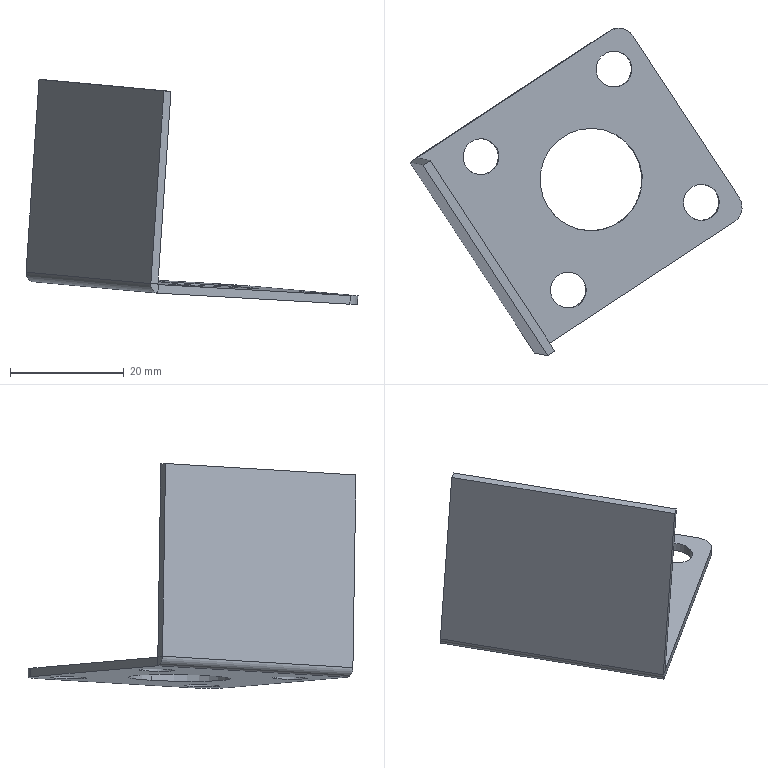Component | SolidWorks | DoorCylinderMount-1 | 1 solid | 26 faces | box 58.28 x 57.54 x 39.49 mm | volume 4144 mm3 | cylinder 14 | plane 12 | commonest cylinder face diameters 6.3 x8 18 x2 6 x2 0.2 x1 3.2 x1 | material AISI 304
STEP:
#1=CARTESIAN_POINT('',(-3.508,6.476,31.173));
#2=VERTEX_POINT('',#1);
#3=CARTESIAN_POINT('',(-3.372,6.269,31.16));
#4=VERTEX_POINT('',#3);
#5=CARTESIAN_POINT('',(-3.44,6.373,31.167));
#6=DIRECTION('',(0.0675,-0.01553,0.9976));
#7=DIRECTION('',(0.5475,-0.8353,-0.05005));
#8=AXIS2_PLACEMENT_3D('',#5,#6,#7);
#9=CIRCLE('',#8,0.124);
#10=EDGE_CURVE('',#2,#4,#9,.T.);
#11=ORIENTED_EDGE('',*,*,#10,.F.);
#12=CARTESIAN_POINT('',(-3.504,6.476,31.232));
#13=VERTEX_POINT('',#12);
#14=CARTESIAN_POINT('',(-3.504,6.476,31.232));
#15=DIRECTION('',(0.0675,-0.01553,0.9976));
#16=VECTOR('',#15,39.37);
#17=LINE('',#14,#16);
#18=EDGE_CURVE('',#2,#13,#17,.T.);
#19=ORIENTED_EDGE('',*,*,#18,.T.);
#20=CARTESIAN_POINT('',(-3.368,6.268,31.219));
#21=VERTEX_POINT('',#20);
#22=CARTESIAN_POINT('',(-3.436,6.372,31.225));
#23=DIRECTION('',(0.0675,-0.01553,0.9976));
#24=DIRECTION('',(0.5475,-0.8353,-0.05005));
#25=AXIS2_PLACEMENT_3D('',#22,#23,#24);
#26=CIRCLE('',#25,0.124);
#27=EDGE_CURVE('',#13,#21,#26,.T.);
#28=ORIENTED_EDGE('',*,*,#27,.T.);
#29=CARTESIAN_POINT('',(-3.368,6.268,31.219));
#30=DIRECTION('',(0.0675,-0.01553,0.9976));
#31=VECTOR('',#30,39.37);
#32=LINE('',#29,#31);
#33=EDGE_CURVE('',#4,#21,#32,.T.);
#34=ORIENTED_EDGE('',*,*,#33,.F.);
#35=EDGE_LOOP('',(#11,#19,#28,#34));
#36=FACE_OUTER_BOUND('',#35,.T.);
#37=CARTESIAN_POINT('',(-3.436,6.372,31.225));
#38=DIRECTION('',(0.0675,-0.01553,0.9976));
#39=DIRECTION('',(0.5475,-0.8353,-0.05005));
#40=AXIS2_PLACEMENT_3D('',#37,#38,#39);
#41=CYLINDRICAL_SURFACE('',#40,0.124);
#42=ADVANCED_FACE('',(#36),#41,.F.);
#43=CARTESIAN_POINT('',(-2.904,5.556,31.118));
#44=VERTEX_POINT('',#43);
#45=CARTESIAN_POINT('',(-2.769,5.348,31.105));
#46=VERTEX_POINT('',#45);
#47=CARTESIAN_POINT('',(-2.837,5.452,31.111));
#48=DIRECTION('',(0.0675,-0.01553,0.9976));
#49=DIRECTION('',(0.5475,-0.8353,-0.05005));
#50=AXIS2_PLACEMENT_3D('',#47,#48,#49);
#51=CIRCLE('',#50,0.124);
#52=EDGE_CURVE('',#44,#46,#51,.T.);
#53=ORIENTED_EDGE('',*,*,#52,.F.);
#54=CARTESIAN_POINT('',(-2.9,5.555,31.176));
#55=VERTEX_POINT('',#54);
#56=CARTESIAN_POINT('',(-2.9,5.555,31.176));
#57=DIRECTION('',(0.0675,-0.01553,0.9976));
#58=VECTOR('',#57,39.37);
#59=LINE('',#56,#58);
#60=EDGE_CURVE('',#44,#55,#59,.T.);
#61=ORIENTED_EDGE('',*,*,#60,.T.);
#62=CARTESIAN_POINT('',(-2.765,5.348,31.164));
#63=VERTEX_POINT('',#62);
#64=CARTESIAN_POINT('',(-2.833,5.451,31.17));
#65=DIRECTION('',(0.0675,-0.01553,0.9976));
#66=DIRECTION('',(0.5475,-0.8353,-0.05005));
#67=AXIS2_PLACEMENT_3D('',#64,#65,#66);
#68=CIRCLE('',#67,0.124);
#69=EDGE_CURVE('',#55,#63,#68,.T.);
#70=ORIENTED_EDGE('',*,*,#69,.T.);
#71=CARTESIAN_POINT('',(-2.765,5.348,31.164));
#72=DIRECTION('',(0.0675,-0.01553,0.9976));
#73=VECTOR('',#72,39.37);
#74=LINE('',#71,#73);
#75=EDGE_CURVE('',#46,#63,#74,.T.);
#76=ORIENTED_EDGE('',*,*,#75,.F.);
#77=EDGE_LOOP('',(#53,#61,#70,#76));
#78=FACE_OUTER_BOUND('',#77,.T.);
#79=CARTESIAN_POINT('',(-2.833,5.451,31.17));
#80=DIRECTION('',(0.0675,-0.01553,0.9976));
#81=DIRECTION('',(0.5475,-0.8353,-0.05005));
#82=AXIS2_PLACEMENT_3D('',#79,#80,#81);
#83=CYLINDRICAL_SURFACE('',#82,0.124);
#84=ADVANCED_FACE('',(#78),#83,.F.);
#85=CARTESIAN_POINT('',(-3.824,4.95,31.17));
#86=VERTEX_POINT('',#85);
#87=CARTESIAN_POINT('',(-3.688,4.743,31.158));
#88=VERTEX_POINT('',#87);
#89=CARTESIAN_POINT('',(-3.756,4.846,31.164));
#90=DIRECTION('',(0.0675,-0.01553,0.9976));
#91=DIRECTION('',(0.5475,-0.8353,-0.05005));
#92=AXIS2_PLACEMENT_3D('',#89,#90,#91);
#93=CIRCLE('',#92,0.124);
#94=EDGE_CURVE('',#86,#88,#93,.T.);
#95=ORIENTED_EDGE('',*,*,#94,.F.);
#96=CARTESIAN_POINT('',(-3.82,4.949,31.229));
#97=VERTEX_POINT('',#96);
#98=CARTESIAN_POINT('',(-3.82,4.949,31.229));
#99=DIRECTION('',(0.0675,-0.01553,0.9976));
#100=VECTOR('',#99,39.37);
#101=LINE('',#98,#100);
#102=EDGE_CURVE('',#86,#97,#101,.T.);
#103=ORIENTED_EDGE('',*,*,#102,.T.);
#104=CARTESIAN_POINT('',(-3.684,4.742,31.217));
#105=VERTEX_POINT('',#104);
#106=CARTESIAN_POINT('',(-3.752,4.845,31.223));
#107=DIRECTION('',(0.0675,-0.01553,0.9976));
#108=DIRECTION('',(0.5475,-0.8353,-0.05005));
#109=AXIS2_PLACEMENT_3D('',#106,#107,#108);
#110=CIRCLE('',#109,0.124);
#111=EDGE_CURVE('',#97,#105,#110,.T.);
#112=ORIENTED_EDGE('',*,*,#111,.T.);
#113=CARTESIAN_POINT('',(-3.684,4.742,31.217));
#114=DIRECTION('',(0.0675,-0.01553,0.9976));
#115=VECTOR('',#114,39.37);
#116=LINE('',#113,#115);
#117=EDGE_CURVE('',#88,#105,#116,.T.);
#118=ORIENTED_EDGE('',*,*,#117,.F.);
#119=EDGE_LOOP('',(#95,#103,#112,#118));
#120=FACE_OUTER_BOUND('',#119,.T.);
#121=CARTESIAN_POINT('',(-3.752,4.845,31.223));
#122=DIRECTION('',(0.0675,-0.01553,0.9976));
#123=DIRECTION('',(0.5475,-0.8353,-0.05005));
#124=AXIS2_PLACEMENT_3D('',#121,#122,#123);
#125=CYLINDRICAL_SURFACE('',#124,0.124);
#126=ADVANCED_FACE('',(#120),#125,.F.);
#127=CARTESIAN_POINT('',(-4.427,5.871,31.226));
#128=VERTEX_POINT('',#127);
#129=CARTESIAN_POINT('',(-4.292,5.663,31.213));
#130=VERTEX_POINT('',#129);
#131=CARTESIAN_POINT('',(-4.36,5.767,31.219));
#132=DIRECTION('',(0.0675,-0.01553,0.9976));
#133=DIRECTION('',(0.5475,-0.8353,-0.05005));
#134=AXIS2_PLACEMENT_3D('',#131,#132,#133);
#135=CIRCLE('',#134,0.124);
#136=EDGE_CURVE('',#128,#130,#135,.T.);
#137=ORIENTED_EDGE('',*,*,#136,.F.);
#138=CARTESIAN_POINT('',(-4.423,5.87,31.284));
#139=VERTEX_POINT('',#138);
#140=CARTESIAN_POINT('',(-4.423,5.87,31.284));
#141=DIRECTION('',(0.0675,-0.01553,0.9976));
#142=VECTOR('',#141,39.37);
#143=LINE('',#140,#142);
#144=EDGE_CURVE('',#128,#139,#143,.T.);
#145=ORIENTED_EDGE('',*,*,#144,.T.);
#146=CARTESIAN_POINT('',(-4.288,5.662,31.272));
#147=VERTEX_POINT('',#146);
#148=CARTESIAN_POINT('',(-4.356,5.766,31.278));
#149=DIRECTION('',(0.0675,-0.01553,0.9976));
#150=DIRECTION('',(0.5475,-0.8353,-0.05005));
#151=AXIS2_PLACEMENT_3D('',#148,#149,#150);
#152=CIRCLE('',#151,0.124);
#153=EDGE_CURVE('',#139,#147,#152,.T.);
#154=ORIENTED_EDGE('',*,*,#153,.T.);
#155=CARTESIAN_POINT('',(-4.288,5.662,31.272));
#156=DIRECTION('',(0.0675,-0.01553,0.9976));
#157=VECTOR('',#156,39.37);
#158=LINE('',#155,#157);
#159=EDGE_CURVE('',#130,#147,#158,.T.);
#160=ORIENTED_EDGE('',*,*,#159,.F.);
#161=EDGE_LOOP('',(#137,#145,#154,#160));
#162=FACE_OUTER_BOUND('',#161,.T.);
#163=CARTESIAN_POINT('',(-4.356,5.766,31.278));
#164=DIRECTION('',(0.0675,-0.01553,0.9976));
#165=DIRECTION('',(0.5475,-0.8353,-0.05005));
#166=AXIS2_PLACEMENT_3D('',#163,#164,#165);
#167=CYLINDRICAL_SURFACE('',#166,0.124);
#168=ADVANCED_FACE('',(#162),#167,.F.);
#169=CARTESIAN_POINT('',(-3.894,5.415,31.182));
#170=VERTEX_POINT('',#169);
#171=CARTESIAN_POINT('',(-3.302,5.804,31.148));
#172=VERTEX_POINT('',#171);
#173=CARTESIAN_POINT('',(-3.598,5.61,31.165));
#174=DIRECTION('',(0.0675,-0.01553,0.9976));
#175=DIRECTION('',(0.8341,0.5496,-0.04788));
#176=AXIS2_PLACEMENT_3D('',#173,#174,#175);
#177=CIRCLE('',#176,0.3543);
#178=EDGE_CURVE('',#170,#172,#177,.T.);
#179=ORIENTED_EDGE('',*,*,#178,.F.);
#180=CARTESIAN_POINT('',(-3.89,5.414,31.241));
#181=VERTEX_POINT('',#180);
#182=CARTESIAN_POINT('',(-3.89,5.414,31.241));
#183=DIRECTION('',(0.0675,-0.01553,0.9976));
#184=VECTOR('',#183,39.37);
#185=LINE('',#182,#184);
#186=EDGE_CURVE('',#170,#181,#185,.T.);
#187=ORIENTED_EDGE('',*,*,#186,.T.);
#188=CARTESIAN_POINT('',(-3.298,5.803,31.207));
#189=VERTEX_POINT('',#188);
#190=CARTESIAN_POINT('',(-3.594,5.609,31.224));
#191=DIRECTION('',(0.0675,-0.01553,0.9976));
#192=DIRECTION('',(0.8341,0.5496,-0.04788));
#193=AXIS2_PLACEMENT_3D('',#190,#191,#192);
#194=CIRCLE('',#193,0.3543);
#195=EDGE_CURVE('',#181,#189,#194,.T.);
#196=ORIENTED_EDGE('',*,*,#195,.T.);
#197=CARTESIAN_POINT('',(-3.298,5.803,31.207));
#198=DIRECTION('',(0.0675,-0.01553,0.9976));
#199=VECTOR('',#198,39.37);
#200=LINE('',#197,#199);
#201=EDGE_CURVE('',#172,#189,#200,.T.);
#202=ORIENTED_EDGE('',*,*,#201,.F.);
#203=EDGE_LOOP('',(#179,#187,#196,#202));
#204=FACE_OUTER_BOUND('',#203,.T.);
#205=CARTESIAN_POINT('',(-3.594,5.609,31.224));
#206=DIRECTION('',(0.0675,-0.01553,0.9976));
#207=DIRECTION('',(0.8341,0.5496,-0.04788));
#208=AXIS2_PLACEMENT_3D('',#205,#206,#207);
#209=CYLINDRICAL_SURFACE('',#208,0.3543);
#210=ADVANCED_FACE('',(#204),#209,.F.);
#211=CARTESIAN_POINT('',(-3.935,4.446,31.17));
#212=VERTEX_POINT('',#211);
#213=CARTESIAN_POINT('',(-2.609,5.32,31.094));
#214=VERTEX_POINT('',#213);
#215=CARTESIAN_POINT('',(-2.51,5.385,31.088));
#216=DIRECTION('',(0.8341,0.5496,-0.04788));
#217=VECTOR('',#216,39.37);
#218=LINE('',#215,#217);
#219=EDGE_CURVE('',#212,#214,#218,.T.);
#220=ORIENTED_EDGE('',*,*,#219,.T.);
#221=CARTESIAN_POINT('',(-2.605,5.319,31.153));
#222=VERTEX_POINT('',#221);
#223=CARTESIAN_POINT('',(-2.605,5.319,31.153));
#224=DIRECTION('',(0.0675,-0.01553,0.9976));
#225=VECTOR('',#224,39.37);
#226=LINE('',#223,#225);
#227=EDGE_CURVE('',#214,#222,#226,.T.);
#228=ORIENTED_EDGE('',*,*,#227,.T.);
#229=CARTESIAN_POINT('',(-3.931,4.445,31.229));
#230=VERTEX_POINT('',#229);
#231=CARTESIAN_POINT('',(-2.506,5.384,31.147));
#232=DIRECTION('',(0.8341,0.5496,-0.04788));
#233=VECTOR('',#232,39.37);
#234=LINE('',#231,#233);
#235=EDGE_CURVE('',#230,#222,#234,.T.);
#236=ORIENTED_EDGE('',*,*,#235,.F.);
#237=CARTESIAN_POINT('',(-3.931,4.445,31.229));
#238=DIRECTION('',(0.0675,-0.01553,0.9976));
#239=VECTOR('',#238,39.37);
#240=LINE('',#237,#239);
#241=EDGE_CURVE('',#212,#230,#240,.T.);
#242=ORIENTED_EDGE('',*,*,#241,.F.);
#243=EDGE_LOOP('',(#220,#228,#236,#242));
#244=FACE_OUTER_BOUND('',#243,.T.);
#245=CARTESIAN_POINT('',(-2.506,5.384,31.147));
#246=DIRECTION('',(-0.5475,0.8353,0.05005));
#247=DIRECTION('',(0.8341,0.5496,-0.04788));
#248=AXIS2_PLACEMENT_3D('',#245,#246,#247);
#249=PLANE('',#248);
#250=ADVANCED_FACE('',(#244),#249,.F.);
#251=CARTESIAN_POINT('',(-3.308,6.601,31.161));
#252=VERTEX_POINT('',#251);
#253=CARTESIAN_POINT('',(-2.575,5.483,31.094));
#254=VERTEX_POINT('',#253);
#255=CARTESIAN_POINT('',(-3.372,6.7,31.167));
#256=DIRECTION('',(0.5475,-0.8353,-0.05005));
#257=VECTOR('',#256,39.37);
#258=LINE('',#255,#257);
#259=EDGE_CURVE('',#252,#254,#258,.T.);
#260=ORIENTED_EDGE('',*,*,#259,.F.);
#261=CARTESIAN_POINT('',(-3.304,6.6,31.22));
#262=VERTEX_POINT('',#261);
#263=CARTESIAN_POINT('',(-3.304,6.6,31.22));
#264=DIRECTION('',(0.0675,-0.01553,0.9976));
#265=VECTOR('',#264,39.37);
#266=LINE('',#263,#265);
#267=EDGE_CURVE('',#252,#262,#266,.T.);
#268=ORIENTED_EDGE('',*,*,#267,.T.);
#269=CARTESIAN_POINT('',(-2.571,5.482,31.153));
#270=VERTEX_POINT('',#269);
#271=CARTESIAN_POINT('',(-3.368,6.699,31.226));
#272=DIRECTION('',(0.5475,-0.8353,-0.05005));
#273=VECTOR('',#272,39.37);
#274=LINE('',#271,#273);
#275=EDGE_CURVE('',#262,#270,#274,.T.);
#276=ORIENTED_EDGE('',*,*,#275,.T.);
#277=CARTESIAN_POINT('',(-2.571,5.482,31.153));
#278=DIRECTION('',(-0.0675,0.01553,-0.9976));
#279=VECTOR('',#278,39.37);
#280=LINE('',#277,#279);
#281=EDGE_CURVE('',#270,#254,#280,.T.);
#282=ORIENTED_EDGE('',*,*,#281,.T.);
#283=EDGE_LOOP('',(#260,#268,#276,#282));
#284=FACE_OUTER_BOUND('',#283,.T.);
#285=CARTESIAN_POINT('',(-3.368,6.699,31.226));
#286=DIRECTION('',(0.8341,0.5496,-0.04788));
#287=DIRECTION('',(0.5475,-0.8353,-0.05005));
#288=AXIS2_PLACEMENT_3D('',#285,#286,#287);
#289=PLANE('',#288);
#290=ADVANCED_FACE('',(#284),#289,.T.);
#291=CARTESIAN_POINT('',(-4.794,5.76,31.308));
#292=VERTEX_POINT('',#291);
#293=CARTESIAN_POINT('',(-3.467,6.634,31.232));
#294=VERTEX_POINT('',#293);
#295=CARTESIAN_POINT('',(-3.368,6.699,31.226));
#296=DIRECTION('',(0.8341,0.5496,-0.04788));
#297=VECTOR('',#296,39.37);
#298=LINE('',#295,#297);
#299=EDGE_CURVE('',#292,#294,#298,.T.);
#300=ORIENTED_EDGE('',*,*,#299,.T.);
#301=CARTESIAN_POINT('',(-3.471,6.635,31.173));
#302=VERTEX_POINT('',#301);
#303=CARTESIAN_POINT('',(-3.467,6.634,31.232));
#304=DIRECTION('',(-0.0675,0.01553,-0.9976));
#305=VECTOR('',#304,39.37);
#306=LINE('',#303,#305);
#307=EDGE_CURVE('',#294,#302,#306,.T.);
#308=ORIENTED_EDGE('',*,*,#307,.T.);
#309=CARTESIAN_POINT('',(-4.798,5.761,31.249));
#310=VERTEX_POINT('',#309);
#311=CARTESIAN_POINT('',(-3.372,6.7,31.167));
#312=DIRECTION('',(0.8341,0.5496,-0.04788));
#313=VECTOR('',#312,39.37);
#314=LINE('',#311,#313);
#315=EDGE_CURVE('',#310,#302,#314,.T.);
#316=ORIENTED_EDGE('',*,*,#315,.F.);
#317=CARTESIAN_POINT('',(-4.794,5.76,31.308));
#318=DIRECTION('',(0.0675,-0.01553,0.9976));
#319=VECTOR('',#318,39.37);
#320=LINE('',#317,#319);
#321=EDGE_CURVE('',#310,#292,#320,.T.);
#322=ORIENTED_EDGE('',*,*,#321,.T.);
#323=EDGE_LOOP('',(#300,#308,#316,#322));
#324=FACE_OUTER_BOUND('',#323,.T.);
#325=CARTESIAN_POINT('',(-3.368,6.699,31.226));
#326=DIRECTION('',(-0.5475,0.8353,0.05005));
#327=DIRECTION('',(0.8341,0.5496,-0.04788));
#328=AXIS2_PLACEMENT_3D('',#325,#326,#327);
#329=PLANE('',#328);
#330=ADVANCED_FACE('',(#324),#329,.T.);
#331=ORIENTED_EDGE('',*,*,#321,.F.);
#332=CARTESIAN_POINT('',(-4.846,5.725,31.315));
#333=VERTEX_POINT('',#332);
#334=CARTESIAN_POINT('',(-4.793,5.76,31.312));
#335=DIRECTION('',(-0.5475,0.8353,0.05005));
#336=DIRECTION('',(0.0675,-0.01553,0.9976));
#337=AXIS2_PLACEMENT_3D('',#334,#335,#336);
#338=CIRCLE('',#337,0.06299);
#339=EDGE_CURVE('',#310,#333,#338,.T.);
#340=ORIENTED_EDGE('',*,*,#339,.T.);
#341=CARTESIAN_POINT('',(-4.797,5.758,31.312));
#342=VERTEX_POINT('',#341);
#343=CARTESIAN_POINT('',(-4.797,5.758,31.312));
#344=DIRECTION('',(0.8341,0.5496,-0.04788));
#345=VECTOR('',#344,39.37);
#346=LINE('',#343,#345);
#347=EDGE_CURVE('',#333,#342,#346,.T.);
#348=ORIENTED_EDGE('',*,*,#347,.T.);
#349=CARTESIAN_POINT('',(-4.793,5.76,31.312));
#350=DIRECTION('',(-0.5475,0.8353,0.05005));
#351=DIRECTION('',(-0.0675,0.01553,-0.9976));
#352=AXIS2_PLACEMENT_3D('',#349,#350,#351);
#353=CIRCLE('',#352,0.003937);
#354=EDGE_CURVE('',#292,#342,#353,.T.);
#355=ORIENTED_EDGE('',*,*,#354,.F.);
#356=EDGE_LOOP('',(#331,#340,#348,#355));
#357=FACE_OUTER_BOUND('',#356,.T.);
#358=CARTESIAN_POINT('',(-4.793,5.76,31.312));
#359=DIRECTION('',(-0.5475,0.8353,0.05005));
#360=DIRECTION('',(0.0675,-0.01553,0.9976));
#361=AXIS2_PLACEMENT_3D('',#358,#359,#360);
#362=PLANE('',#361);
#363=ADVANCED_FACE('',(#357),#362,.T.);
#364=ORIENTED_EDGE('',*,*,#347,.F.);
#365=CARTESIAN_POINT('',(-4.756,5.705,32.646));
#366=VERTEX_POINT('',#365);
#367=CARTESIAN_POINT('',(-4.846,5.725,31.311));
#368=DIRECTION('',(-0.0675,0.01553,-0.9976));
#369=VECTOR('',#368,39.37);
#370=LINE('',#367,#369);
#371=EDGE_CURVE('',#366,#333,#370,.T.);
#372=ORIENTED_EDGE('',*,*,#371,.F.);
#373=CARTESIAN_POINT('',(-4.706,5.737,32.643));
#374=VERTEX_POINT('',#373);
#375=CARTESIAN_POINT('',(-4.706,5.737,32.643));
#376=DIRECTION('',(0.8341,0.5496,-0.04788));
#377=VECTOR('',#376,39.37);
#378=LINE('',#375,#377);
#379=EDGE_CURVE('',#366,#374,#378,.T.);
#380=ORIENTED_EDGE('',*,*,#379,.T.);
#381=CARTESIAN_POINT('',(-4.797,5.758,31.308));
#382=DIRECTION('',(-0.0675,0.01553,-0.9976));
#383=VECTOR('',#382,39.37);
#384=LINE('',#381,#383);
#385=EDGE_CURVE('',#374,#342,#384,.T.);
#386=ORIENTED_EDGE('',*,*,#385,.T.);
#387=EDGE_LOOP('',(#364,#372,#380,#386));
#388=FACE_OUTER_BOUND('',#387,.T.);
#389=CARTESIAN_POINT('',(-4.797,5.758,31.308));
#390=DIRECTION('',(-0.5475,0.8353,0.05005));
#391=DIRECTION('',(-0.0675,0.01553,-0.9976));
#392=AXIS2_PLACEMENT_3D('',#389,#390,#391);
#393=PLANE('',#392);
#394=ADVANCED_FACE('',(#388),#393,.T.);
#395=ORIENTED_EDGE('',*,*,#379,.F.);
#396=CARTESIAN_POINT('',(-3.893,4.389,32.567));
#397=VERTEX_POINT('',#396);
#398=CARTESIAN_POINT('',(-4.756,5.705,32.646));
#399=DIRECTION('',(0.5475,-0.8353,-0.05005));
#400=VECTOR('',#399,39.37);
#401=LINE('',#398,#400);
#402=EDGE_CURVE('',#366,#397,#401,.T.);
#403=ORIENTED_EDGE('',*,*,#402,.T.);
#404=CARTESIAN_POINT('',(-3.844,4.422,32.565));
#405=VERTEX_POINT('',#404);
#406=CARTESIAN_POINT('',(-3.844,4.422,32.565));
#407=DIRECTION('',(0.8341,0.5496,-0.04788));
#408=VECTOR('',#407,39.37);
#409=LINE('',#406,#408);
#410=EDGE_CURVE('',#397,#405,#409,.T.);
#411=ORIENTED_EDGE('',*,*,#410,.T.);
#412=CARTESIAN_POINT('',(-4.706,5.737,32.643));
#413=DIRECTION('',(0.5475,-0.8353,-0.05005));
#414=VECTOR('',#413,39.37);
#415=LINE('',#412,#414);
#416=EDGE_CURVE('',#374,#405,#415,.T.);
#417=ORIENTED_EDGE('',*,*,#416,.F.);
#418=EDGE_LOOP('',(#395,#403,#411,#417));
#419=FACE_OUTER_BOUND('',#418,.T.);
#420=CARTESIAN_POINT('',(-4.706,5.737,32.643));
#421=DIRECTION('',(-0.0675,0.01553,-0.9976));
#422=DIRECTION('',(0.5475,-0.8353,-0.05005));
#423=AXIS2_PLACEMENT_3D('',#420,#421,#422);
#424=PLANE('',#423);
#425=ADVANCED_FACE('',(#419),#424,.F.);
#426=ORIENTED_EDGE('',*,*,#410,.F.);
#427=CARTESIAN_POINT('',(-3.984,4.41,31.236));
#428=VERTEX_POINT('',#427);
#429=CARTESIAN_POINT('',(-3.984,4.41,31.232));
#430=DIRECTION('',(-0.0675,0.01553,-0.9976));
#431=VECTOR('',#430,39.37);
#432=LINE('',#429,#431);
#433=EDGE_CURVE('',#397,#428,#432,.T.);
#434=ORIENTED_EDGE('',*,*,#433,.T.);
#435=CARTESIAN_POINT('',(-3.934,4.442,31.233));
#436=VERTEX_POINT('',#435);
#437=CARTESIAN_POINT('',(-3.934,4.442,31.233));
#438=DIRECTION('',(0.8341,0.5496,-0.04788));
#439=VECTOR('',#438,39.37);
#440=LINE('',#437,#439);
#441=EDGE_CURVE('',#428,#436,#440,.T.);
#442=ORIENTED_EDGE('',*,*,#441,.T.);
#443=CARTESIAN_POINT('',(-3.935,4.442,31.229));
#444=DIRECTION('',(-0.0675,0.01553,-0.9976));
#445=VECTOR('',#444,39.37);
#446=LINE('',#443,#445);
#447=EDGE_CURVE('',#405,#436,#446,.T.);
#448=ORIENTED_EDGE('',*,*,#447,.F.);
#449=EDGE_LOOP('',(#426,#434,#442,#448));
#450=FACE_OUTER_BOUND('',#449,.T.);
#451=CARTESIAN_POINT('',(-3.935,4.442,31.229));
#452=DIRECTION('',(-0.5475,0.8353,0.05005));
#453=DIRECTION('',(-0.0675,0.01553,-0.9976));
#454=AXIS2_PLACEMENT_3D('',#451,#452,#453);
#455=PLANE('',#454);
#456=ADVANCED_FACE('',(#450),#455,.F.);
#457=ORIENTED_EDGE('',*,*,#186,.F.);
#458=CARTESIAN_POINT('',(-3.598,5.61,31.165));
#459=DIRECTION('',(0.0675,-0.01553,0.9976));
#460=DIRECTION('',(0.8341,0.5496,-0.04788));
#461=AXIS2_PLACEMENT_3D('',#458,#459,#460);
#462=CIRCLE('',#461,0.3543);
#463=EDGE_CURVE('',#172,#170,#462,.T.);
#464=ORIENTED_EDGE('',*,*,#463,.F.);
#465=ORIENTED_EDGE('',*,*,#201,.T.);
#466=CARTESIAN_POINT('',(-3.594,5.609,31.224));
#467=DIRECTION('',(0.0675,-0.01553,0.9976));
#468=DIRECTION('',(0.8341,0.5496,-0.04788));
#469=AXIS2_PLACEMENT_3D('',#466,#467,#468);
#470=CIRCLE('',#469,0.3543);
#471=EDGE_CURVE('',#189,#181,#470,.T.);
#472=ORIENTED_EDGE('',*,*,#471,.T.);
#473=EDGE_LOOP('',(#457,#464,#465,#472));
#474=FACE_OUTER_BOUND('',#473,.T.);
#475=CARTESIAN_POINT('',(-3.594,5.609,31.224));
#476=DIRECTION('',(0.0675,-0.01553,0.9976));
#477=DIRECTION('',(0.8341,0.5496,-0.04788));
#478=AXIS2_PLACEMENT_3D('',#475,#476,#477);
#479=CYLINDRICAL_SURFACE('',#478,0.3543);
#480=ADVANCED_FACE('',(#474),#479,.F.);
#481=ORIENTED_EDGE('',*,*,#144,.F.);
#482=CARTESIAN_POINT('',(-4.36,5.767,31.219));
#483=DIRECTION('',(0.0675,-0.01553,0.9976));
#484=DIRECTION('',(0.5475,-0.8353,-0.05005));
#485=AXIS2_PLACEMENT_3D('',#482,#483,#484);
#486=CIRCLE('',#485,0.124);
#487=EDGE_CURVE('',#130,#128,#486,.T.);
#488=ORIENTED_EDGE('',*,*,#487,.F.);
#489=ORIENTED_EDGE('',*,*,#159,.T.);
#490=CARTESIAN_POINT('',(-4.356,5.766,31.278));
#491=DIRECTION('',(0.0675,-0.01553,0.9976));
#492=DIRECTION('',(0.5475,-0.8353,-0.05005));
#493=AXIS2_PLACEMENT_3D('',#490,#491,#492);
#494=CIRCLE('',#493,0.124);
#495=EDGE_CURVE('',#147,#139,#494,.T.);
#496=ORIENTED_EDGE('',*,*,#495,.T.);
#497=EDGE_LOOP('',(#481,#488,#489,#496));
#498=FACE_OUTER_BOUND('',#497,.T.);
#499=CARTESIAN_POINT('',(-4.356,5.766,31.278));
#500=DIRECTION('',(0.0675,-0.01553,0.9976));
#501=DIRECTION('',(0.5475,-0.8353,-0.05005));
#502=AXIS2_PLACEMENT_3D('',#499,#500,#501);
#503=CYLINDRICAL_SURFACE('',#502,0.124);
#504=ADVANCED_FACE('',(#498),#503,.F.);
#505=ORIENTED_EDGE('',*,*,#102,.F.);
#506=CARTESIAN_POINT('',(-3.756,4.846,31.164));
#507=DIRECTION('',(0.0675,-0.01553,0.9976));
#508=DIRECTION('',(0.5475,-0.8353,-0.05005));
#509=AXIS2_PLACEMENT_3D('',#506,#507,#508);
#510=CIRCLE('',#509,0.124);
#511=EDGE_CURVE('',#88,#86,#510,.T.);
#512=ORIENTED_EDGE('',*,*,#511,.F.);
#513=ORIENTED_EDGE('',*,*,#117,.T.);
#514=CARTESIAN_POINT('',(-3.752,4.845,31.223));
#515=DIRECTION('',(0.0675,-0.01553,0.9976));
#516=DIRECTION('',(0.5475,-0.8353,-0.05005));
#517=AXIS2_PLACEMENT_3D('',#514,#515,#516);
#518=CIRCLE('',#517,0.124);
#519=EDGE_CURVE('',#105,#97,#518,.T.);
#520=ORIENTED_EDGE('',*,*,#519,.T.);
#521=EDGE_LOOP('',(#505,#512,#513,#520));
#522=FACE_OUTER_BOUND('',#521,.T.);
#523=CARTESIAN_POINT('',(-3.752,4.845,31.223));
#524=DIRECTION('',(0.0675,-0.01553,0.9976));
#525=DIRECTION('',(0.5475,-0.8353,-0.05005));
#526=AXIS2_PLACEMENT_3D('',#523,#524,#525);
#527=CYLINDRICAL_SURFACE('',#526,0.124);
#528=ADVANCED_FACE('',(#522),#527,.F.);
#529=ORIENTED_EDGE('',*,*,#60,.F.);
#530=CARTESIAN_POINT('',(-2.837,5.452,31.111));
#531=DIRECTION('',(0.0675,-0.01553,0.9976));
#532=DIRECTION('',(0.5475,-0.8353,-0.05005));
#533=AXIS2_PLACEMENT_3D('',#530,#531,#532);
#534=CIRCLE('',#533,0.124);
#535=EDGE_CURVE('',#46,#44,#534,.T.);
#536=ORIENTED_EDGE('',*,*,#535,.F.);
#537=ORIENTED_EDGE('',*,*,#75,.T.);
#538=CARTESIAN_POINT('',(-2.833,5.451,31.17));
#539=DIRECTION('',(0.0675,-0.01553,0.9976));
#540=DIRECTION('',(0.5475,-0.8353,-0.05005));
#541=AXIS2_PLACEMENT_3D('',#538,#539,#540);
#542=CIRCLE('',#541,0.124);
#543=EDGE_CURVE('',#63,#55,#542,.T.);
#544=ORIENTED_EDGE('',*,*,#543,.T.);
#545=EDGE_LOOP('',(#529,#536,#537,#544));
#546=FACE_OUTER_BOUND('',#545,.T.);
#547=CARTESIAN_POINT('',(-2.833,5.451,31.17));
#548=DIRECTION('',(0.0675,-0.01553,0.9976));
#549=DIRECTION('',(0.5475,-0.8353,-0.05005));
#550=AXIS2_PLACEMENT_3D('',#547,#548,#549);
#551=CYLINDRICAL_SURFACE('',#550,0.124);
#552=ADVANCED_FACE('',(#546),#551,.F.);
#553=ORIENTED_EDGE('',*,*,#18,.F.);
#554=CARTESIAN_POINT('',(-3.44,6.373,31.167));
#555=DIRECTION('',(0.0675,-0.01553,0.9976));
#556=DIRECTION('',(0.5475,-0.8353,-0.05005));
#557=AXIS2_PLACEMENT_3D('',#554,#555,#556);
#558=CIRCLE('',#557,0.124);
#559=EDGE_CURVE('',#4,#2,#558,.T.);
#560=ORIENTED_EDGE('',*,*,#559,.F.);
#561=ORIENTED_EDGE('',*,*,#33,.T.);
#562=CARTESIAN_POINT('',(-3.436,6.372,31.225));
#563=DIRECTION('',(0.0675,-0.01553,0.9976));
#564=DIRECTION('',(0.5475,-0.8353,-0.05005));
#565=AXIS2_PLACEMENT_3D('',#562,#563,#564);
#566=CIRCLE('',#565,0.124);
#567=EDGE_CURVE('',#21,#13,#566,.T.);
#568=ORIENTED_EDGE('',*,*,#567,.T.);
#569=EDGE_LOOP('',(#553,#560,#561,#568));
#570=FACE_OUTER_BOUND('',#569,.T.);
#571=CARTESIAN_POINT('',(-3.436,6.372,31.225));
#572=DIRECTION('',(0.0675,-0.01553,0.9976));
#573=DIRECTION('',(0.5475,-0.8353,-0.05005));
#574=AXIS2_PLACEMENT_3D('',#571,#572,#573);
#575=CYLINDRICAL_SURFACE('',#574,0.124);
#576=ADVANCED_FACE('',(#570),#575,.F.);
#577=CARTESIAN_POINT('',(-3.931,4.445,31.233));
#578=DIRECTION('',(0.5475,-0.8353,-0.05005));
#579=DIRECTION('',(0.0675,-0.01553,0.9976));
#580=AXIS2_PLACEMENT_3D('',#577,#578,#579);
#581=CIRCLE('',#580,0.06299);
#582=EDGE_CURVE('',#428,#212,#581,.T.);
#583=ORIENTED_EDGE('',*,*,#582,.T.);
#584=ORIENTED_EDGE('',*,*,#241,.T.);
#585=CARTESIAN_POINT('',(-3.931,4.445,31.233));
#586=DIRECTION('',(0.5475,-0.8353,-0.05005));
#587=DIRECTION('',(0.0675,-0.01553,0.9976));
#588=AXIS2_PLACEMENT_3D('',#585,#586,#587);
#589=CIRCLE('',#588,0.003937);
#590=EDGE_CURVE('',#436,#230,#589,.T.);
#591=ORIENTED_EDGE('',*,*,#590,.F.);
#592=ORIENTED_EDGE('',*,*,#441,.F.);
#593=EDGE_LOOP('',(#583,#584,#591,#592));
#594=FACE_OUTER_BOUND('',#593,.T.);
#595=CARTESIAN_POINT('',(-3.931,4.445,31.233));
#596=DIRECTION('',(0.5475,-0.8353,-0.05005));
#597=DIRECTION('',(-0.0675,0.01553,-0.9976));
#598=AXIS2_PLACEMENT_3D('',#595,#596,#597);
#599=PLANE('',#598);
#600=ADVANCED_FACE('',(#594),#599,.T.);
#601=ORIENTED_EDGE('',*,*,#447,.T.);
#602=CARTESIAN_POINT('',(-4.797,5.758,31.312));
#603=DIRECTION('',(-0.5475,0.8353,0.05005));
#604=VECTOR('',#603,39.37);
#605=LINE('',#602,#604);
#606=EDGE_CURVE('',#436,#342,#605,.T.);
#607=ORIENTED_EDGE('',*,*,#606,.T.);
#608=ORIENTED_EDGE('',*,*,#385,.F.);
#609=ORIENTED_EDGE('',*,*,#416,.T.);
#610=EDGE_LOOP('',(#601,#607,#608,#609));
#611=FACE_OUTER_BOUND('',#610,.T.);
#612=CARTESIAN_POINT('',(-4.797,5.758,31.308));
#613=DIRECTION('',(-0.8341,-0.5496,0.04788));
#614=DIRECTION('',(0.5475,-0.8353,-0.05005));
#615=AXIS2_PLACEMENT_3D('',#612,#613,#614);
#616=PLANE('',#615);
#617=ADVANCED_FACE('',(#611),#616,.F.);
#618=ORIENTED_EDGE('',*,*,#471,.F.);
#619=ORIENTED_EDGE('',*,*,#195,.F.);
#620=EDGE_LOOP('',(#618,#619));
#621=FACE_BOUND('',#620,.T.);
#622=ORIENTED_EDGE('',*,*,#495,.F.);
#623=ORIENTED_EDGE('',*,*,#153,.F.);
#624=EDGE_LOOP('',(#622,#623));
#625=FACE_BOUND('',#624,.T.);
#626=ORIENTED_EDGE('',*,*,#519,.F.);
#627=ORIENTED_EDGE('',*,*,#111,.F.);
#628=EDGE_LOOP('',(#626,#627));
#629=FACE_BOUND('',#628,.T.);
#630=ORIENTED_EDGE('',*,*,#543,.F.);
#631=ORIENTED_EDGE('',*,*,#69,.F.);
#632=EDGE_LOOP('',(#630,#631));
#633=FACE_BOUND('',#632,.T.);
#634=ORIENTED_EDGE('',*,*,#567,.F.);
#635=ORIENTED_EDGE('',*,*,#27,.F.);
#636=EDGE_LOOP('',(#634,#635));
#637=FACE_BOUND('',#636,.T.);
#638=ORIENTED_EDGE('',*,*,#275,.F.);
#639=CARTESIAN_POINT('',(-3.402,6.535,31.226));
#640=DIRECTION('',(0.0675,-0.01553,0.9976));
#641=DIRECTION('',(-0.8341,-0.5496,0.04788));
#642=AXIS2_PLACEMENT_3D('',#639,#640,#641);
#643=CIRCLE('',#642,0.1181);
#644=EDGE_CURVE('',#262,#294,#643,.T.);
#645=ORIENTED_EDGE('',*,*,#644,.T.);
#646=ORIENTED_EDGE('',*,*,#299,.F.);
#647=CARTESIAN_POINT('',(-3.931,4.445,31.229));
#648=DIRECTION('',(0.5475,-0.8353,-0.05005));
#649=VECTOR('',#648,39.37);
#650=LINE('',#647,#649);
#651=EDGE_CURVE('',#292,#230,#650,.T.);
#652=ORIENTED_EDGE('',*,*,#651,.T.);
#653=ORIENTED_EDGE('',*,*,#235,.T.);
#654=CARTESIAN_POINT('',(-2.669,5.417,31.159));
#655=DIRECTION('',(0.0675,-0.01553,0.9976));
#656=DIRECTION('',(-0.8341,-0.5496,0.04788));
#657=AXIS2_PLACEMENT_3D('',#654,#655,#656);
#658=CIRCLE('',#657,0.1181);
#659=EDGE_CURVE('',#222,#270,#658,.T.);
#660=ORIENTED_EDGE('',*,*,#659,.T.);
#661=EDGE_LOOP('',(#638,#645,#646,#652,#653,#660));
#662=FACE_OUTER_BOUND('',#661,.T.);
#663=CARTESIAN_POINT('',(-3.368,6.699,31.226));
#664=DIRECTION('',(-0.0675,0.01553,-0.9976));
#665=DIRECTION('',(-0.8341,-0.5496,0.04788));
#666=AXIS2_PLACEMENT_3D('',#663,#664,#665);
#667=PLANE('',#666);
#668=ADVANCED_FACE('',(#621,#625,#629,#633,#637,#662),#667,.F.);
#669=ORIENTED_EDGE('',*,*,#354,.T.);
#670=ORIENTED_EDGE('',*,*,#606,.F.);
#671=ORIENTED_EDGE('',*,*,#590,.T.);
#672=ORIENTED_EDGE('',*,*,#651,.F.);
#673=EDGE_LOOP('',(#669,#670,#671,#672));
#674=FACE_OUTER_BOUND('',#673,.T.);
#675=CARTESIAN_POINT('',(-4.793,5.76,31.312));
#676=DIRECTION('',(-0.5475,0.8353,0.05005));
#677=DIRECTION('',(0.0675,-0.01553,0.9976));
#678=AXIS2_PLACEMENT_3D('',#675,#676,#677);
#679=CYLINDRICAL_SURFACE('',#678,0.003937);
#680=ADVANCED_FACE('',(#674),#679,.F.);
#681=ORIENTED_EDGE('',*,*,#433,.F.);
#682=ORIENTED_EDGE('',*,*,#402,.F.);
#683=ORIENTED_EDGE('',*,*,#371,.T.);
#684=CARTESIAN_POINT('',(-4.846,5.725,31.315));
#685=DIRECTION('',(-0.5475,0.8353,0.05005));
#686=VECTOR('',#685,39.37);
#687=LINE('',#684,#686);
#688=EDGE_CURVE('',#428,#333,#687,.T.);
#689=ORIENTED_EDGE('',*,*,#688,.F.);
#690=EDGE_LOOP('',(#681,#682,#683,#689));
#691=FACE_OUTER_BOUND('',#690,.T.);
#692=CARTESIAN_POINT('',(-4.846,5.725,31.311));
#693=DIRECTION('',(-0.8341,-0.5496,0.04788));
#694=DIRECTION('',(0.5475,-0.8353,-0.05005));
#695=AXIS2_PLACEMENT_3D('',#692,#693,#694);
#696=PLANE('',#695);
#697=ADVANCED_FACE('',(#691),#696,.T.);
#698=ORIENTED_EDGE('',*,*,#463,.T.);
#699=ORIENTED_EDGE('',*,*,#178,.T.);
#700=EDGE_LOOP('',(#698,#699));
#701=FACE_BOUND('',#700,.T.);
#702=ORIENTED_EDGE('',*,*,#487,.T.);
#703=ORIENTED_EDGE('',*,*,#136,.T.);
#704=EDGE_LOOP('',(#702,#703));
#705=FACE_BOUND('',#704,.T.);
#706=ORIENTED_EDGE('',*,*,#511,.T.);
#707=ORIENTED_EDGE('',*,*,#94,.T.);
#708=EDGE_LOOP('',(#706,#707));
#709=FACE_BOUND('',#708,.T.);
#710=ORIENTED_EDGE('',*,*,#535,.T.);
#711=ORIENTED_EDGE('',*,*,#52,.T.);
#712=EDGE_LOOP('',(#710,#711));
#713=FACE_BOUND('',#712,.T.);
#714=ORIENTED_EDGE('',*,*,#559,.T.);
#715=ORIENTED_EDGE('',*,*,#10,.T.);
#716=EDGE_LOOP('',(#714,#715));
#717=FACE_BOUND('',#716,.T.);
#718=ORIENTED_EDGE('',*,*,#315,.T.);
#719=CARTESIAN_POINT('',(-3.406,6.536,31.167));
#720=DIRECTION('',(-0.0675,0.01553,-0.9976));
#721=DIRECTION('',(-0.8341,-0.5496,0.04788));
#722=AXIS2_PLACEMENT_3D('',#719,#720,#721);
#723=CIRCLE('',#722,0.1181);
#724=EDGE_CURVE('',#302,#252,#723,.T.);
#725=ORIENTED_EDGE('',*,*,#724,.T.);
#726=ORIENTED_EDGE('',*,*,#259,.T.);
#727=CARTESIAN_POINT('',(-2.673,5.418,31.1));
#728=DIRECTION('',(-0.0675,0.01553,-0.9976));
#729=DIRECTION('',(-0.8341,-0.5496,0.04788));
#730=AXIS2_PLACEMENT_3D('',#727,#728,#729);
#731=CIRCLE('',#730,0.1181);
#732=EDGE_CURVE('',#254,#214,#731,.T.);
#733=ORIENTED_EDGE('',*,*,#732,.T.);
#734=ORIENTED_EDGE('',*,*,#219,.F.);
#735=CARTESIAN_POINT('',(-4.798,5.761,31.249));
#736=DIRECTION('',(0.5475,-0.8353,-0.05005));
#737=VECTOR('',#736,39.37);
#738=LINE('',#735,#737);
#739=EDGE_CURVE('',#310,#212,#738,.T.);
#740=ORIENTED_EDGE('',*,*,#739,.F.);
#741=EDGE_LOOP('',(#718,#725,#726,#733,#734,#740));
#742=FACE_OUTER_BOUND('',#741,.T.);
#743=CARTESIAN_POINT('',(-3.372,6.7,31.167));
#744=DIRECTION('',(-0.0675,0.01553,-0.9976));
#745=DIRECTION('',(-0.8341,-0.5496,0.04788));
#746=AXIS2_PLACEMENT_3D('',#743,#744,#745);
#747=PLANE('',#746);
#748=ADVANCED_FACE('',(#701,#705,#709,#713,#717,#742),#747,.T.);
#749=ORIENTED_EDGE('',*,*,#339,.F.);
#750=ORIENTED_EDGE('',*,*,#739,.T.);
#751=ORIENTED_EDGE('',*,*,#582,.F.);
#752=ORIENTED_EDGE('',*,*,#688,.T.);
#753=EDGE_LOOP('',(#749,#750,#751,#752));
#754=FACE_OUTER_BOUND('',#753,.T.);
#755=CARTESIAN_POINT('',(-4.793,5.76,31.312));
#756=DIRECTION('',(-0.5475,0.8353,0.05005));
#757=DIRECTION('',(0.0675,-0.01553,0.9976));
#758=AXIS2_PLACEMENT_3D('',#755,#756,#757);
#759=CYLINDRICAL_SURFACE('',#758,0.06299);
#760=ADVANCED_FACE('',(#754),#759,.T.);
#761=ORIENTED_EDGE('',*,*,#724,.F.);
#762=ORIENTED_EDGE('',*,*,#307,.F.);
#763=ORIENTED_EDGE('',*,*,#644,.F.);
#764=ORIENTED_EDGE('',*,*,#267,.F.);
#765=EDGE_LOOP('',(#761,#762,#763,#764));
#766=FACE_OUTER_BOUND('',#765,.T.);
#767=CARTESIAN_POINT('',(-3.402,6.535,31.226));
#768=DIRECTION('',(0.0675,-0.01553,0.9976));
#769=DIRECTION('',(0.8341,0.5496,-0.04788));
#770=AXIS2_PLACEMENT_3D('',#767,#768,#769);
#771=CYLINDRICAL_SURFACE('',#770,0.1181);
#772=ADVANCED_FACE('',(#766),#771,.T.);
#773=ORIENTED_EDGE('',*,*,#732,.F.);
#774=ORIENTED_EDGE('',*,*,#281,.F.);
#775=ORIENTED_EDGE('',*,*,#659,.F.);
#776=ORIENTED_EDGE('',*,*,#227,.F.);
#777=EDGE_LOOP('',(#773,#774,#775,#776));
#778=FACE_OUTER_BOUND('',#777,.T.);
#779=CARTESIAN_POINT('',(-2.669,5.417,31.159));
#780=DIRECTION('',(-0.0675,0.01553,-0.9976));
#781=DIRECTION('',(-0.8341,-0.5496,0.04788));
#782=AXIS2_PLACEMENT_3D('',#779,#780,#781);
#783=CYLINDRICAL_SURFACE('',#782,0.1181);
#784=ADVANCED_FACE('',(#778),#783,.T.);
#785=CLOSED_SHELL('',(#42,#84,#126,#168,#210,#250,#290,#330,#363,#394,#425,#456,#480,#504,#528,#552,#576,#600,#617,#668,#680,#697,#748,#760,#772,#784));
#786=MANIFOLD_SOLID_BREP('',#785);
#787=CARTESIAN_POINT('',(0.,0.,0.));
#788=DIRECTION('',(0.,0.,1.));
#789=DIRECTION('',(1.,0.,0.));
#790=AXIS2_PLACEMENT_3D('',#787,#788,#789);
#791=(LENGTH_UNIT()NAMED_UNIT(*)SI_UNIT($,.METRE.));
#792=LENGTH_MEASURE_WITH_UNIT(LENGTH_MEASURE(0.0254),#791);
#793=DIMENSIONAL_EXPONENTS(1.,0.,0.,0.,0.,0.,0.);
#794=(CONVERSION_BASED_UNIT('',#792)LENGTH_UNIT()NAMED_UNIT(#793));
#795=UNCERTAINTY_MEASURE_WITH_UNIT(LENGTH_MEASURE(0.00001),#794,'','');
#796=(NAMED_UNIT(*)PLANE_ANGLE_UNIT()SI_UNIT($,.RADIAN.));
#797=(NAMED_UNIT(*)SI_UNIT($,.STERADIAN.)SOLID_ANGLE_UNIT());
#798=(GEOMETRIC_REPRESENTATION_CONTEXT(3)GLOBAL_UNCERTAINTY_ASSIGNED_CONTEXT((#795))GLOBAL_UNIT_ASSIGNED_CONTEXT((#794,#796,#797))REPRESENTATION_CONTEXT('',''));
#799=ADVANCED_BREP_SHAPE_REPRESENTATION('',(#786,#790),#798);
#800=COLOUR_RGB('',0.7922,0.8196,0.9333);
#801=FILL_AREA_STYLE_COLOUR('',#800);
#802=FILL_AREA_STYLE('',(#801));
#803=SURFACE_STYLE_FILL_AREA(#802);
#804=SURFACE_SIDE_STYLE('',(#803));
#805=SURFACE_STYLE_USAGE(.BOTH.,#804);
#806=PRESENTATION_STYLE_ASSIGNMENT((#805));
#807=STYLED_ITEM('',(#806),#786);
#808=PRESENTATION_LAYER_ASSIGNMENT('','',(#807));
#809=(LENGTH_UNIT()NAMED_UNIT(*)SI_UNIT($,.METRE.));
#810=LENGTH_MEASURE_WITH_UNIT(LENGTH_MEASURE(0.0254),#809);
#811=DIMENSIONAL_EXPONENTS(1.,0.,0.,0.,0.,0.,0.);
#812=(CONVERSION_BASED_UNIT('',#810)LENGTH_UNIT()NAMED_UNIT(#811));
#813=UNCERTAINTY_MEASURE_WITH_UNIT(LENGTH_MEASURE(0.00001),#812,'','');
#814=(NAMED_UNIT(*)PLANE_ANGLE_UNIT()SI_UNIT($,.RADIAN.));
#815=(NAMED_UNIT(*)SI_UNIT($,.STERADIAN.)SOLID_ANGLE_UNIT());
#816=(GEOMETRIC_REPRESENTATION_CONTEXT(3)GLOBAL_UNCERTAINTY_ASSIGNED_CONTEXT((#813))GLOBAL_UNIT_ASSIGNED_CONTEXT((#812,#814,#815))REPRESENTATION_CONTEXT('',''));
#817=MECHANICAL_DESIGN_GEOMETRIC_PRESENTATION_REPRESENTATION('',(#807),#816);